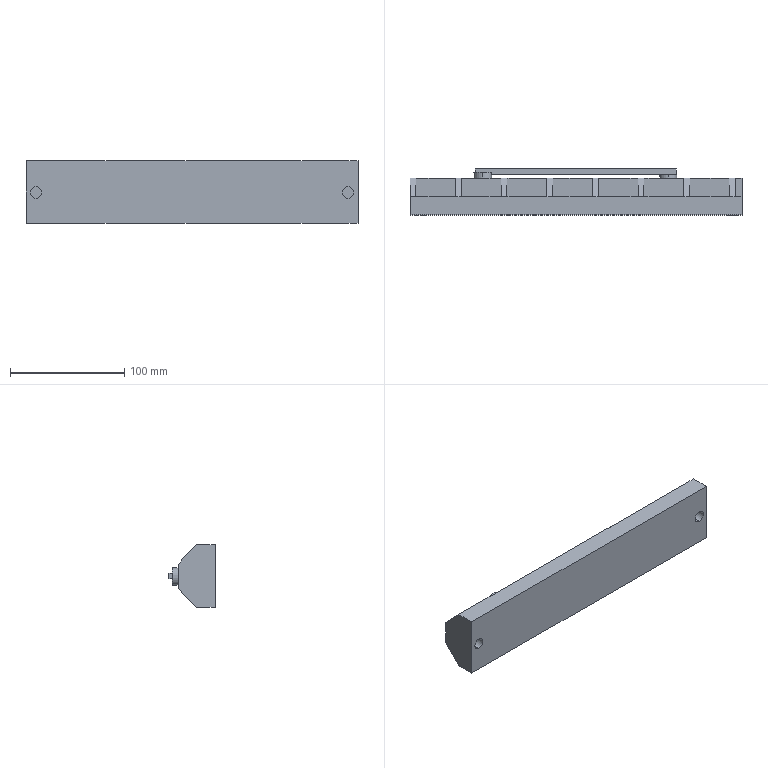Component | SolidWorks | Part20-1 | 1 solid | 104 faces | volume 372713 mm3 | plane 96 | cylinder 8 | commonest cylinder face diameters 10 x4 15 x2 15.519 x2